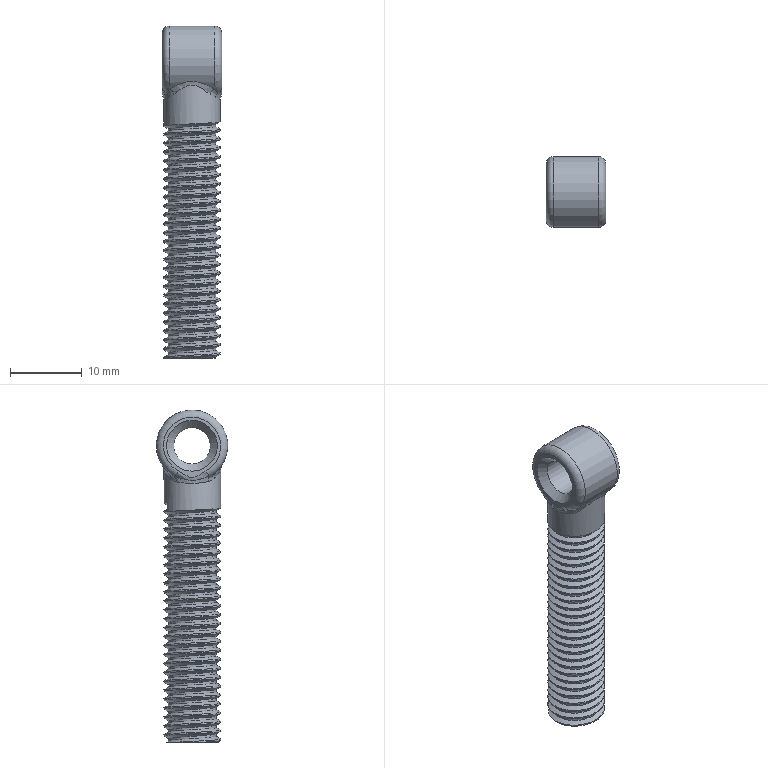Component | NX | BOLT | 1 solid | 49 faces | volume 1986 mm3 | cylinder 29 | spline 12 | plane 4 | cone 2 | torus 2 | commonest cylinder face diameters 7.94 x26 10 x1 5.1 x1 6.69 x1